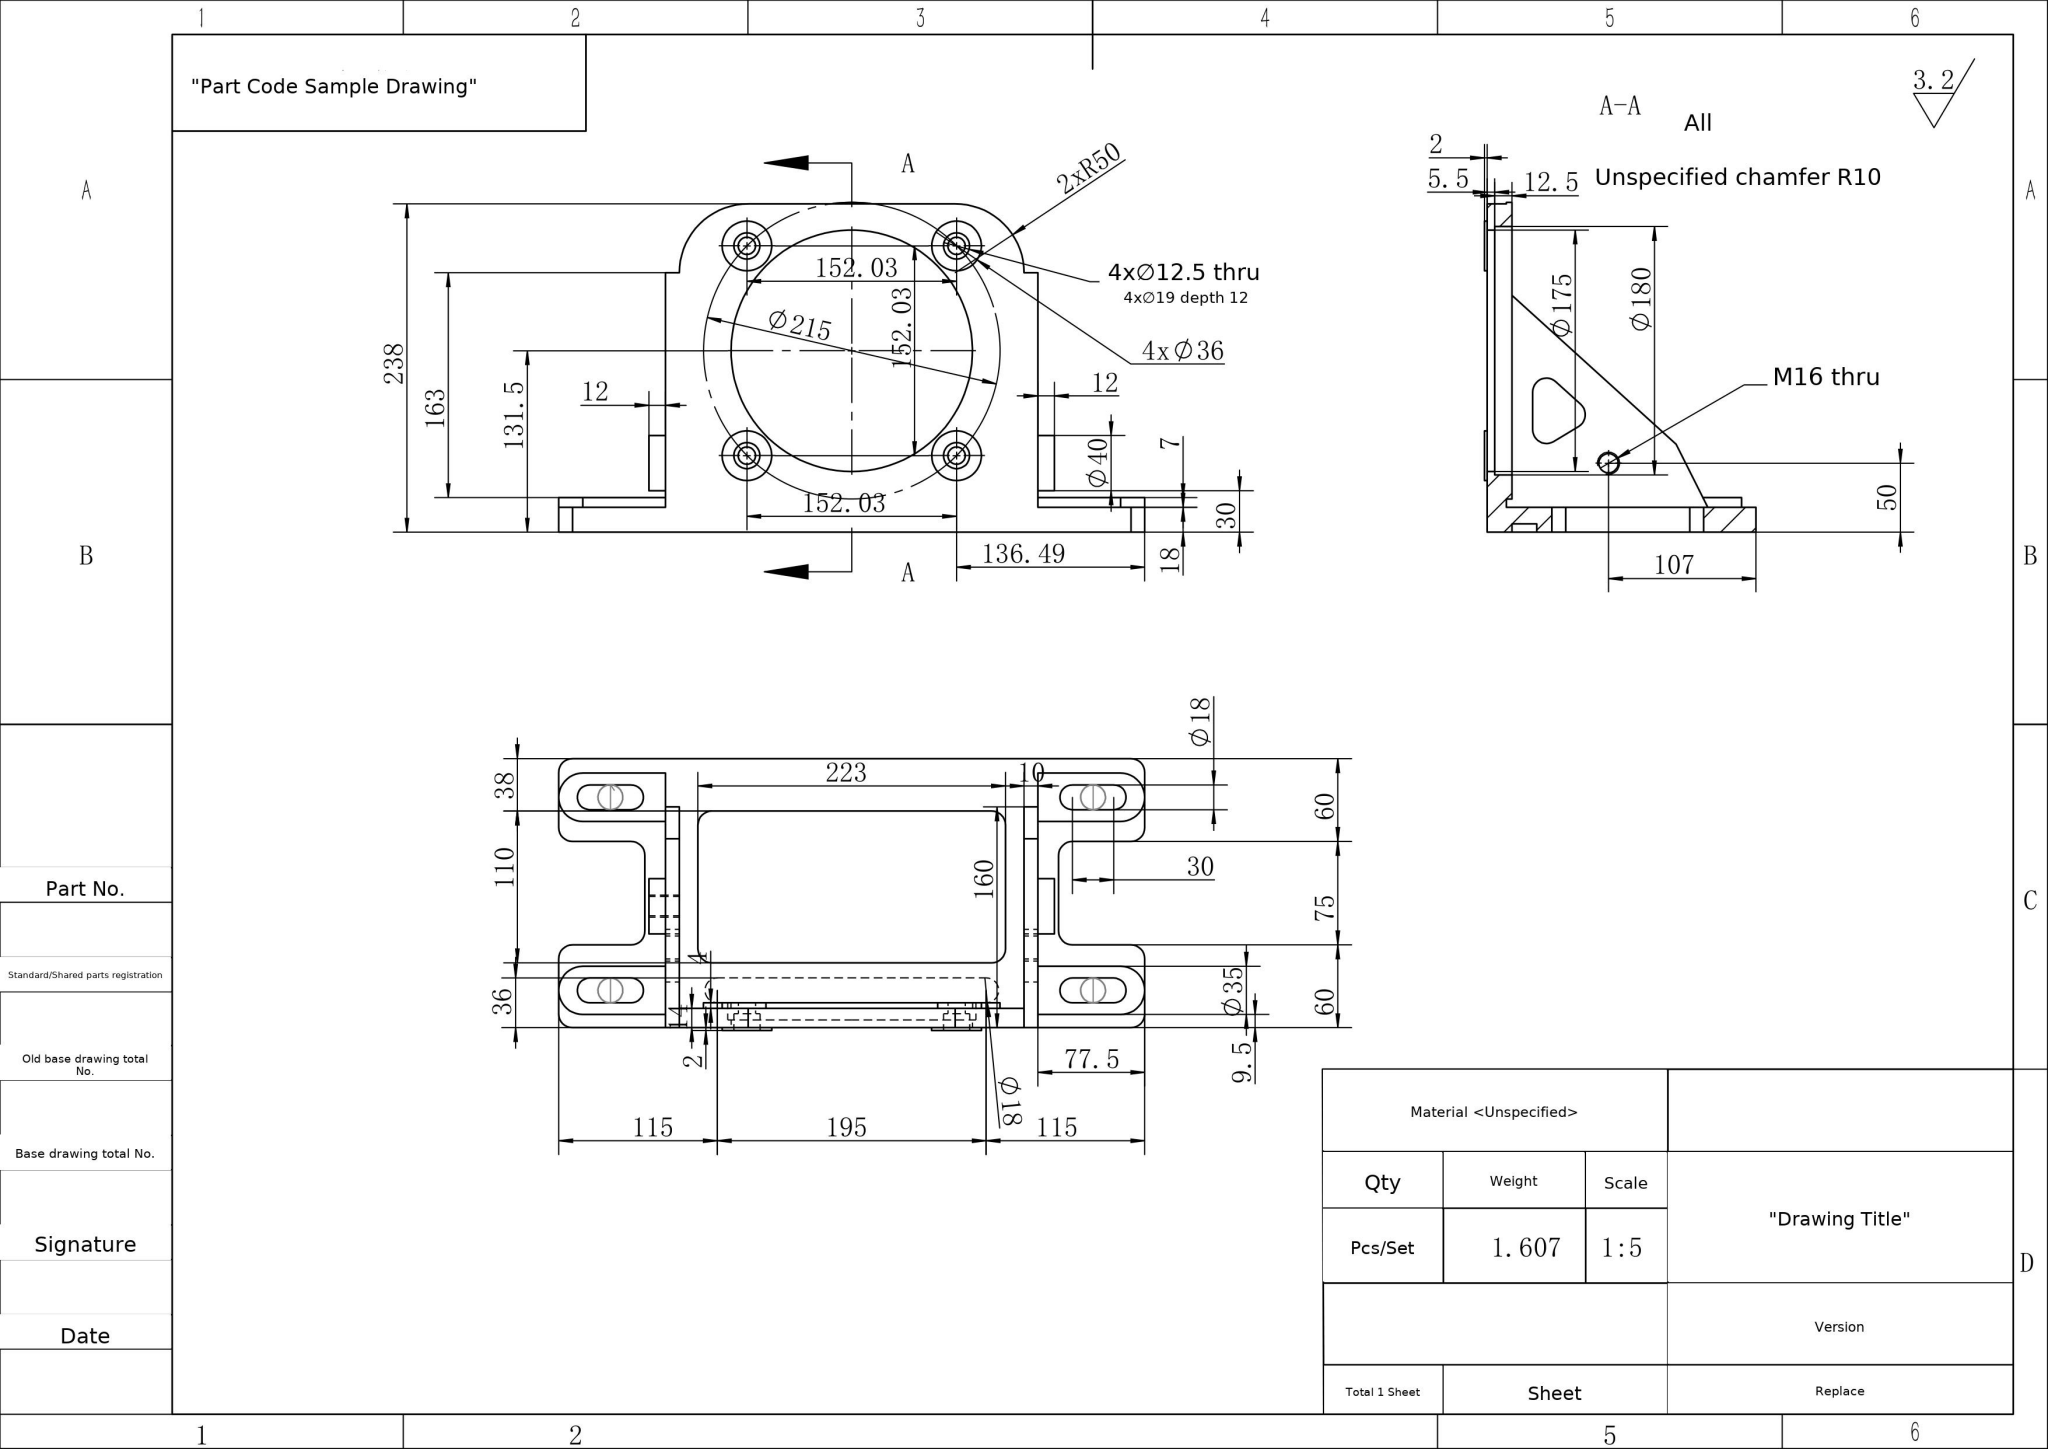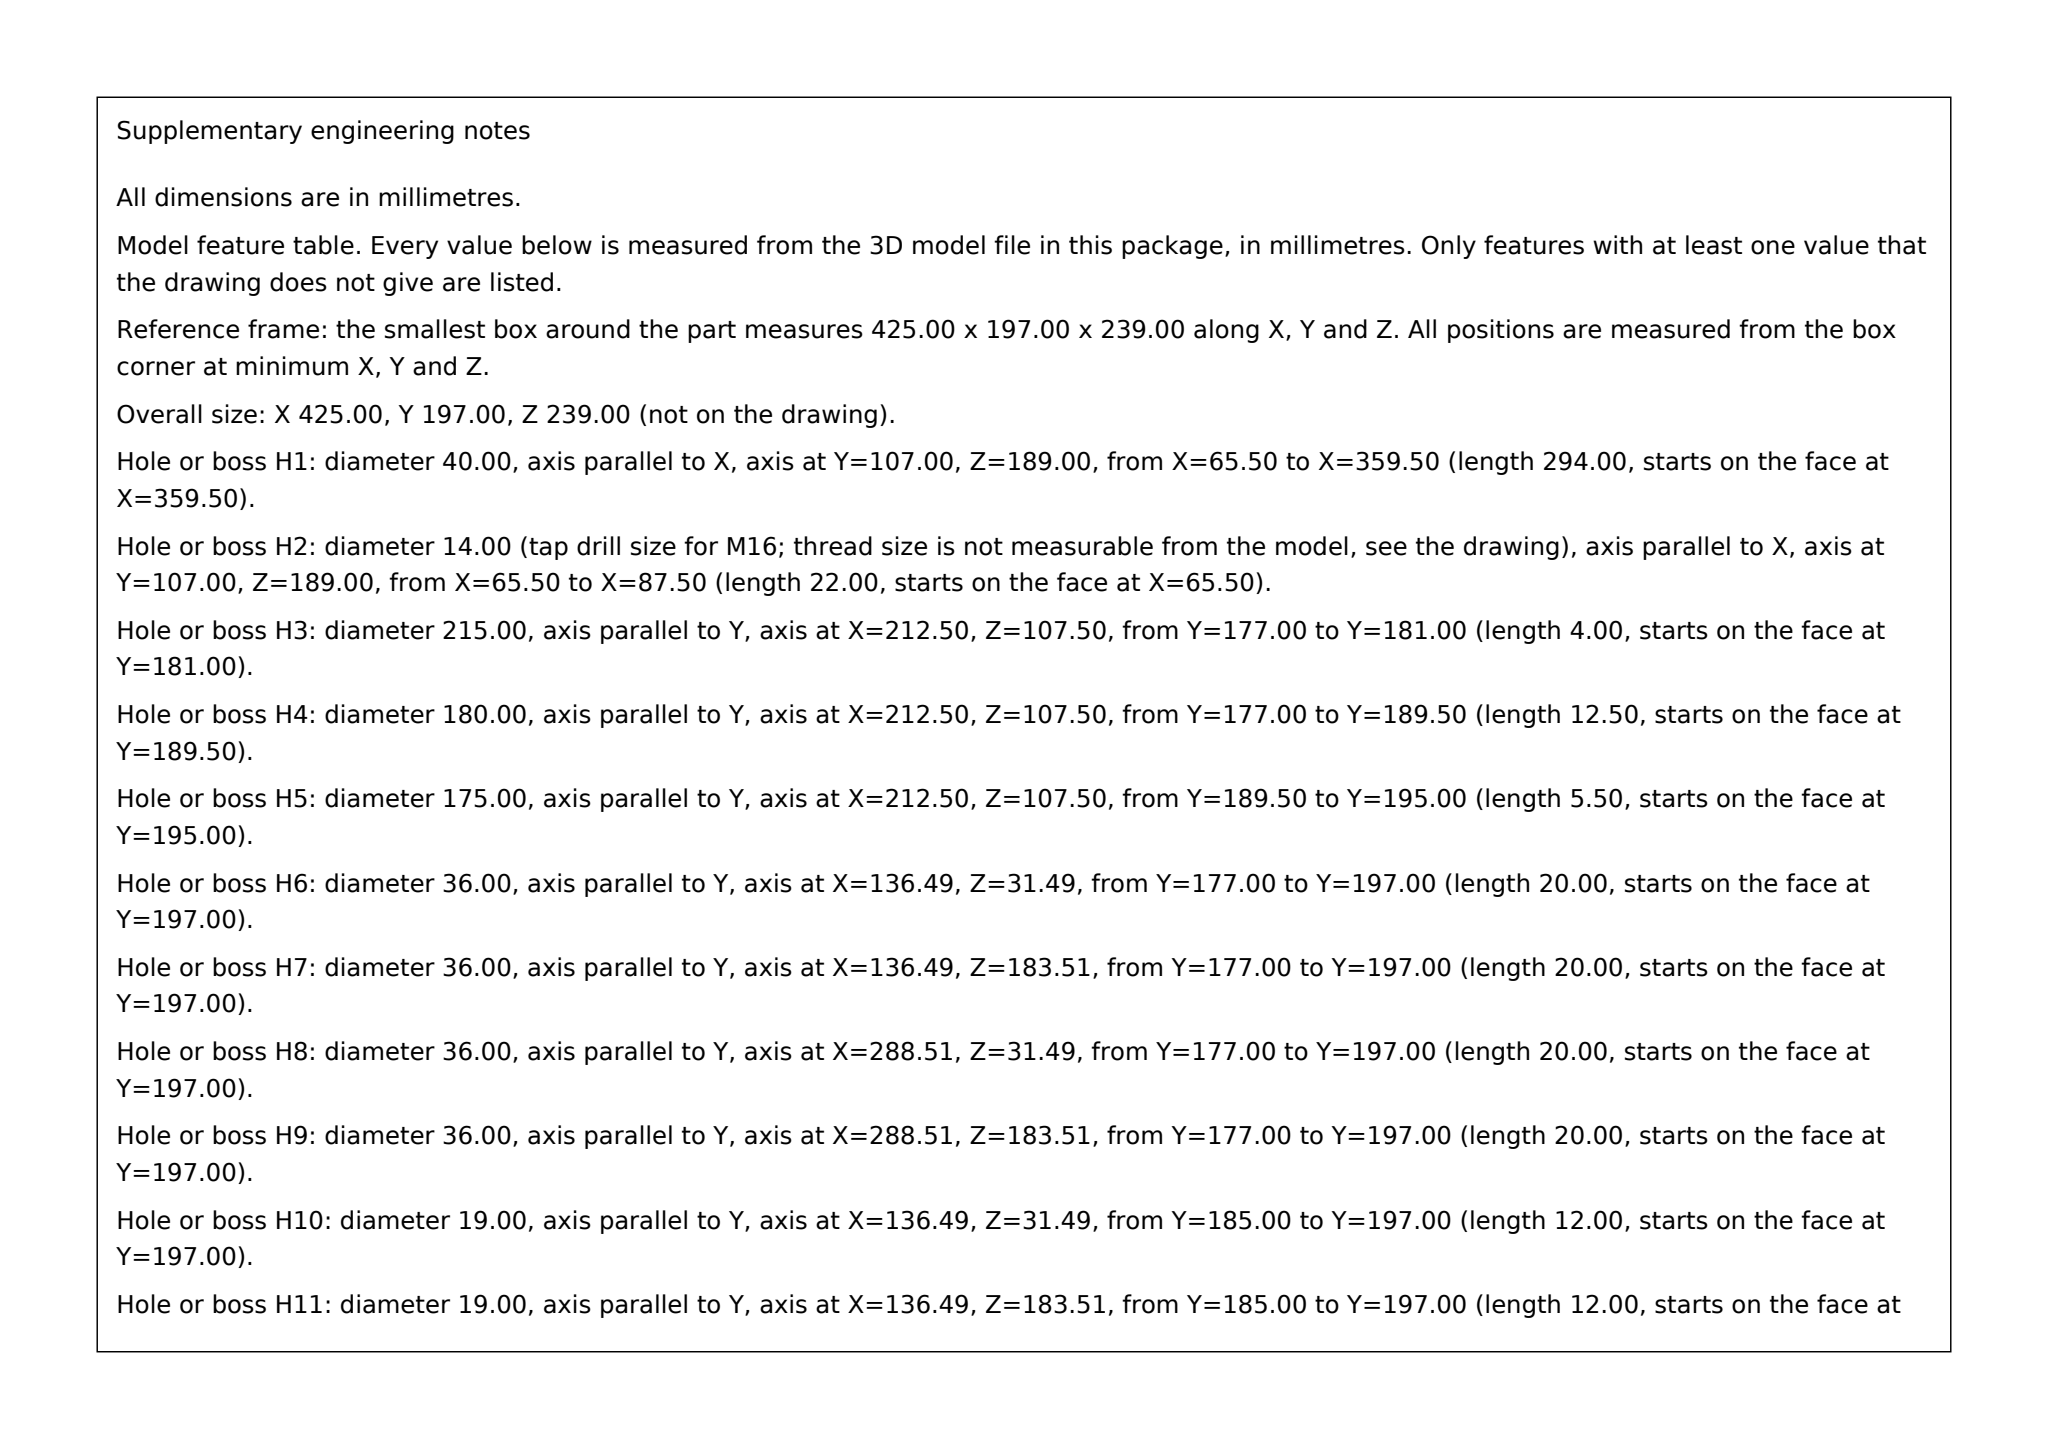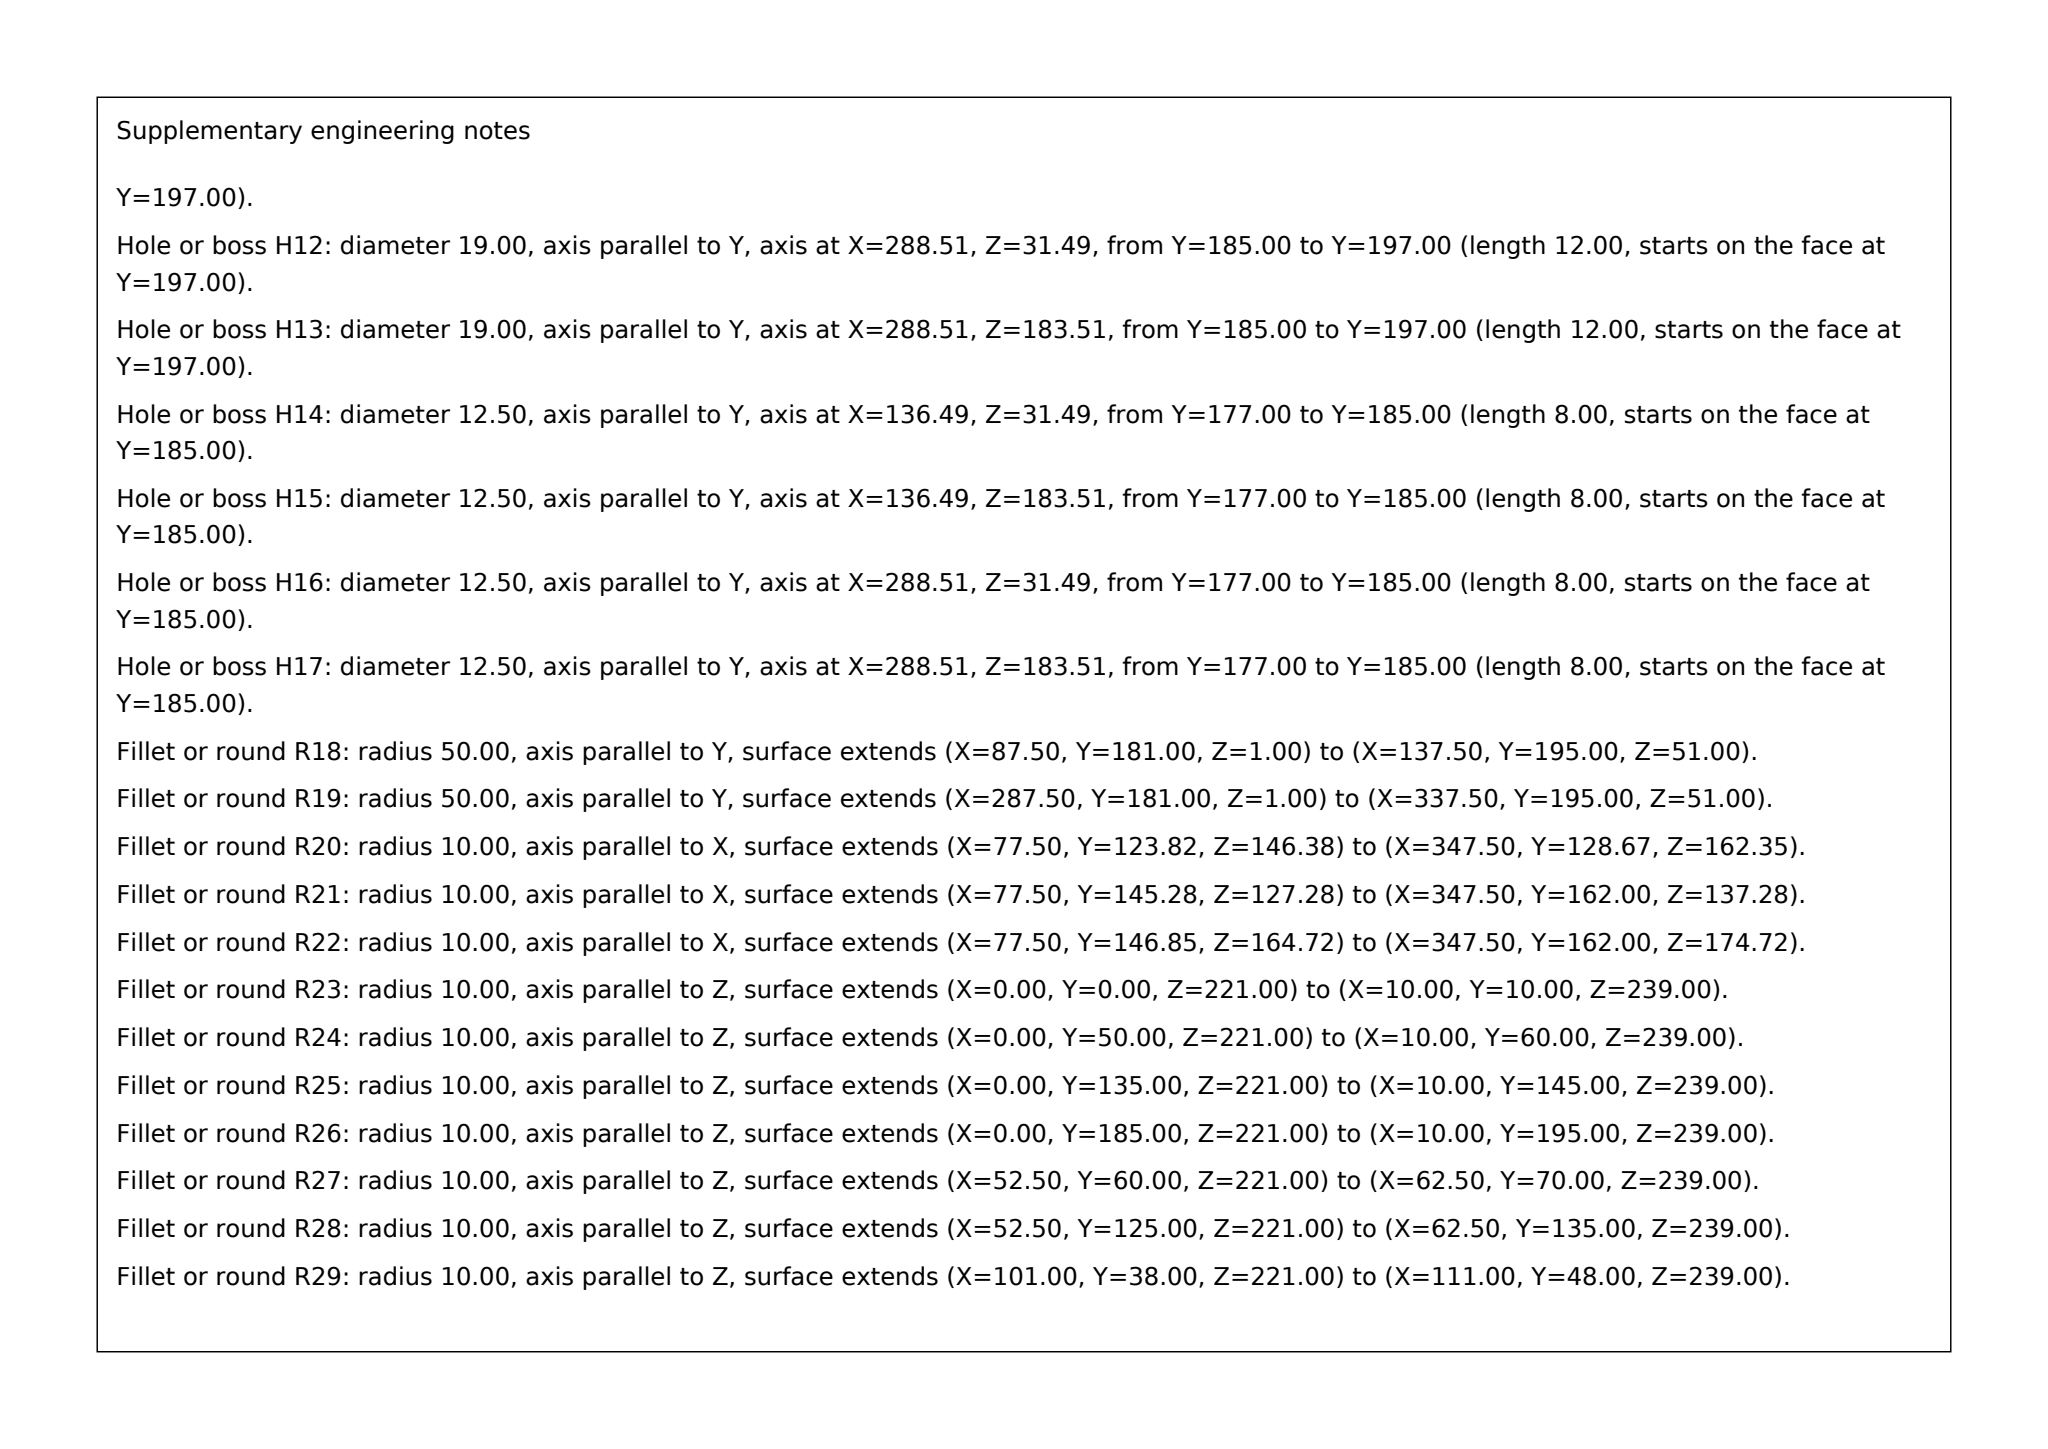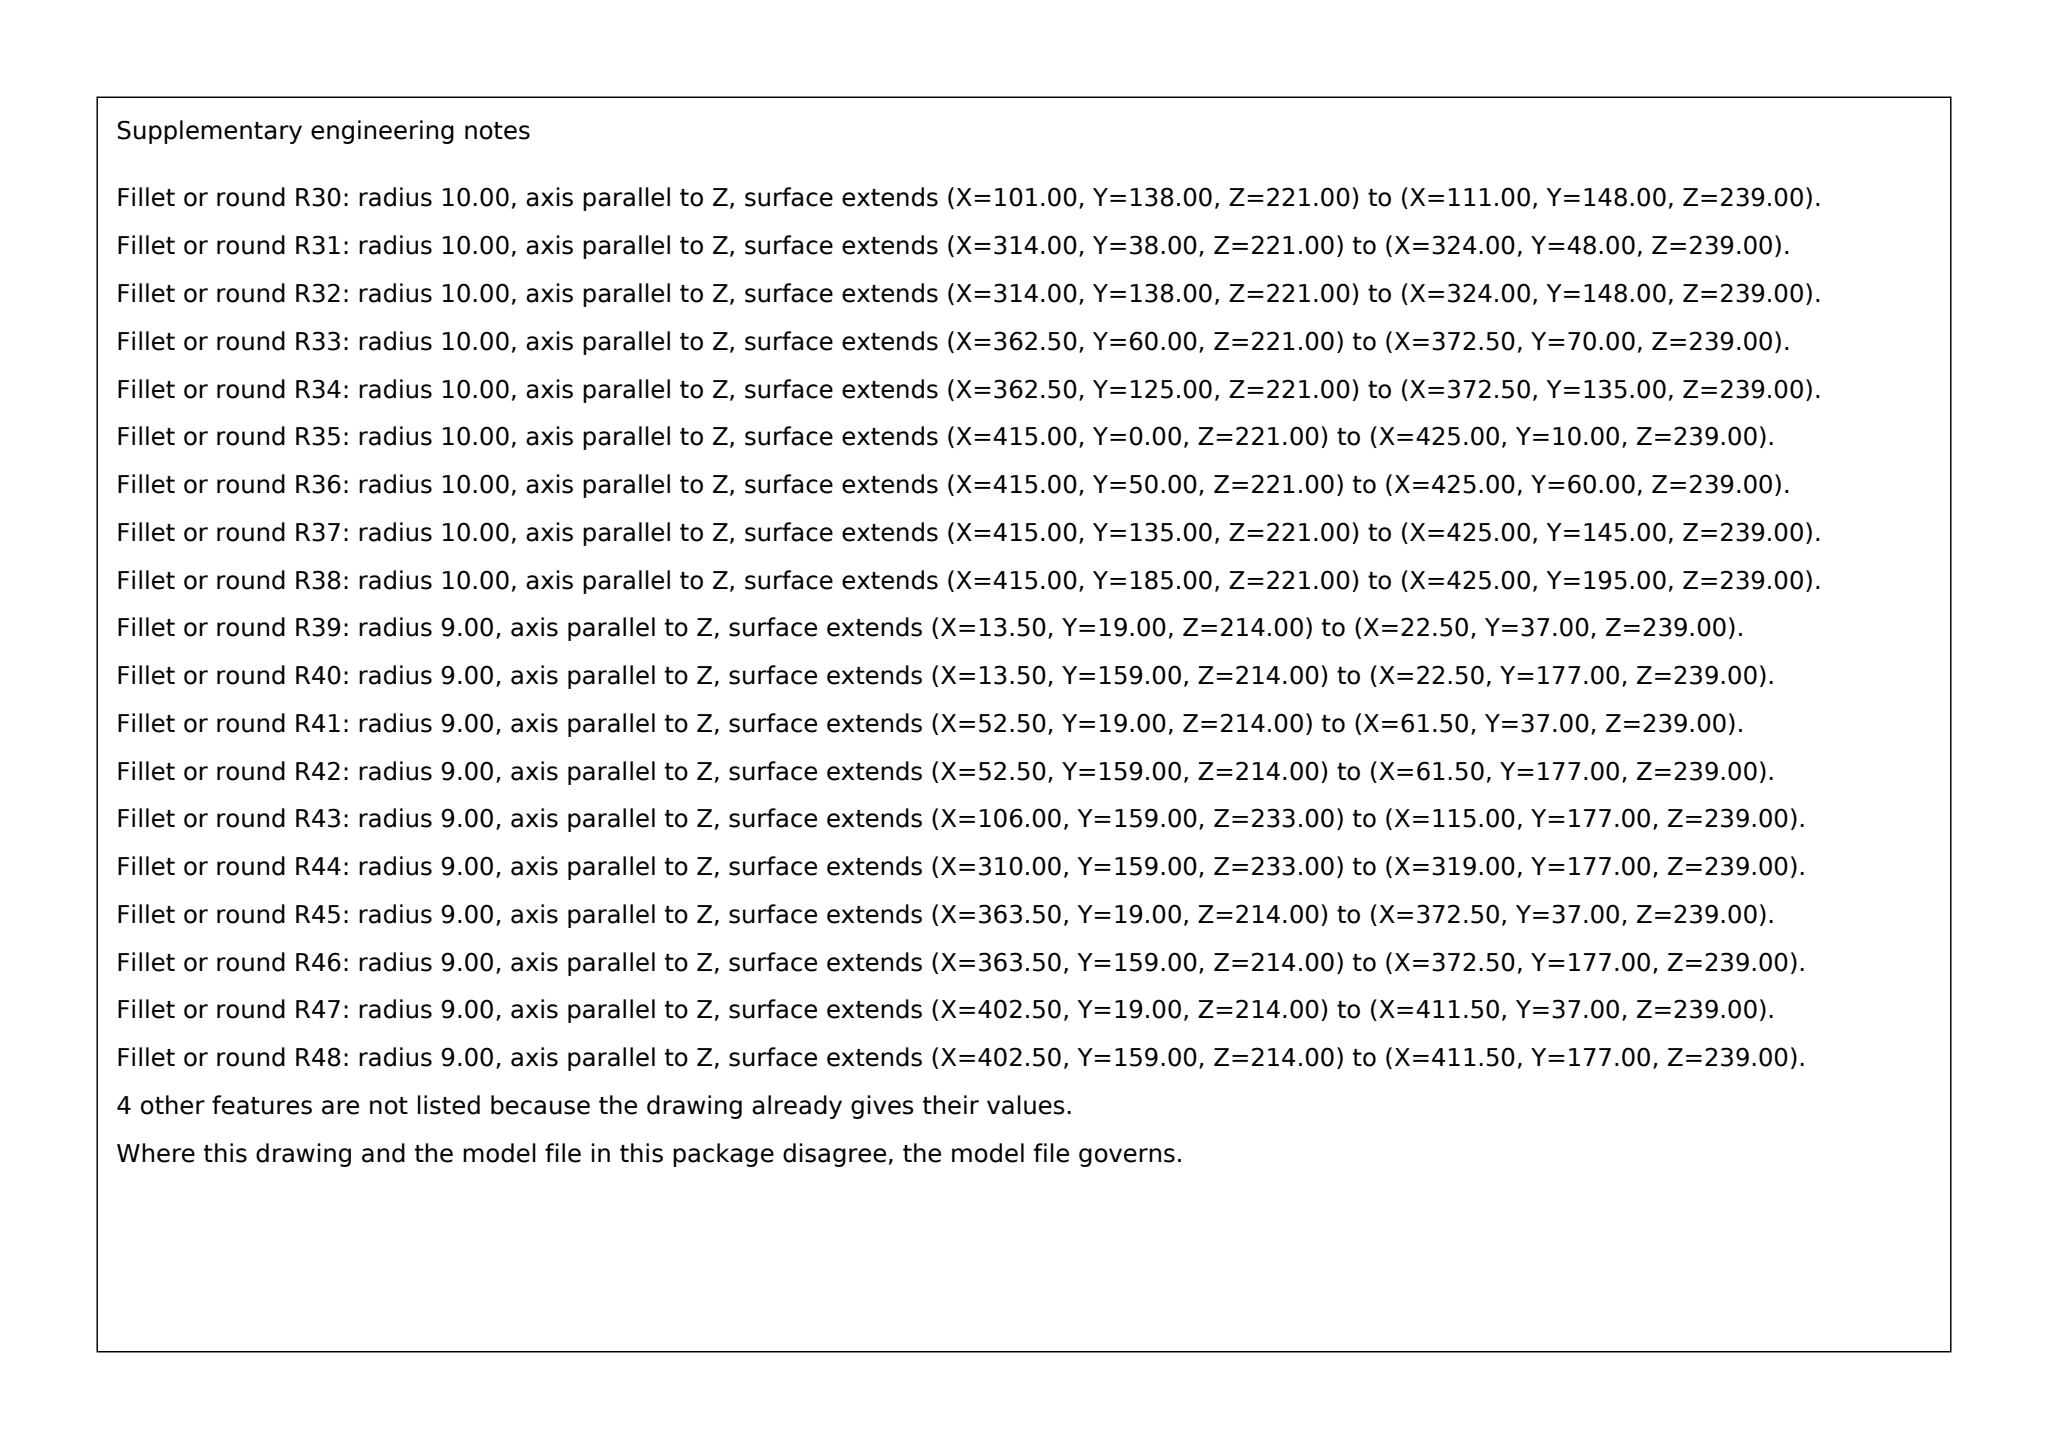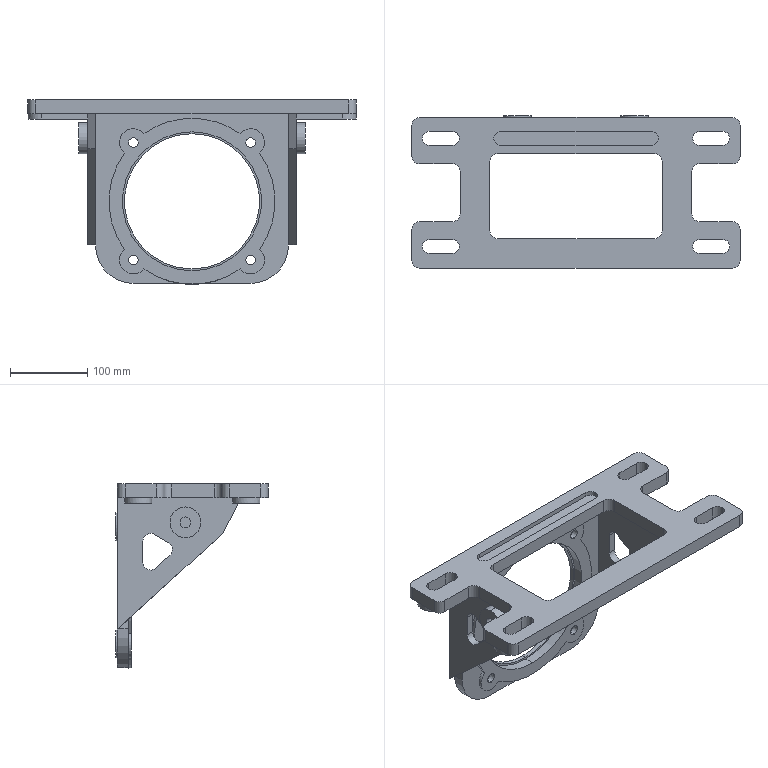Part | SolidWorks | mm | 1 solid | 170 faces | box 425 x 197 x 239 mm | volume 1607400 mm3 | cylinder 92 | plane 78 | commonest cylinder face diameters 20 x24 18 x15 36 x14 12.5 x8 19 x8 35 x6 215 x5 40 x4
build123d program:
from build123d import *

# Parameters (mm, degrees)
SKETCH1_W                    = 223
SKETCH1_H                    = 110
BOSS_EXTRUDE1_DEPTH          = 18
SKETCH2_W                    = 250
SKETCH2_H                    = 220
SKETCH2_R                    = 87.5
BOSS_EXTRUDE2_DEPTH          = 14
SKETCH3_R                    = 90
BOSS_EXTRUDE3_DEPTH          = 4
BOSS_EXTRUDE4_DEPTH          = 10
CUT_EXTRUDE1_START           = -8.5
SKETCH5_R                    = 90
CUT_EXTRUDE1_DEPTH           = 8.5
BOSS_EXTRUDE5_START          = 2
SKETCH6_R                    = 18
BOSS_EXTRUDE5_DEPTH          = 2
SKETCH7_R                    = 9.5
CUT_EXTRUDE2_DEPTH           = 12
F_12_5_12_5_DIAMETER_HOLE1_D = 12.5
BOSS_EXTRUDE6_DEPTH          = 7
FILLET1_R                    = 50
SKETCH11_R                   = 20
BOSS_EXTRUDE7_DEPTH          = 12
M16_TAPPED_HOLE1_D           = 14
M16_TAPPED_HOLE1_DEPTH       = 22
CUT_EXTRUDE4_DEPTH           = 424.671
FILLET2_R                    = 10
FILLET3_R                    = 10
CUT_EXTRUDE5_DEPTH           = 6
CUT_EXTRUDE6_DEPTH           = 335.929


with BuildPart() as part:
    # Sketch1 → Boss-Extrude1 (new body)
    with BuildSketch(Plane.XY):
        Polygon((-212.5, 97.5), (212.5, 97.5), (212.5, 37.5), (150, 37.5), (150, -37.5), (212.5, -37.5), (212.5, -97.5), (-212.5, -97.5), (-212.5, -37.5), (-150, -37.5), (-150, 37.5), (-212.5, 37.5), align=None)
        with Locations((0, -4.5)):
            Rectangle(SKETCH1_W, SKETCH1_H, mode=Mode.SUBTRACT)
    extrude(amount=BOSS_EXTRUDE1_DEPTH)

    # Sketch2 → Boss-Extrude2 (add)
    with BuildSketch(Plane(origin=(0, 97.5, 0), x_dir=(1, 0, 0), z_dir=(0, 1, 0))):
        with Locations((0, 110)):
            Rectangle(SKETCH2_W, SKETCH2_H)
        with Locations(Location((0, 113.5, 0), (0, 0, 270))):
            Circle(SKETCH2_R, mode=Mode.SUBTRACT)
    extrude(amount=-BOSS_EXTRUDE2_DEPTH)

    # Sketch3 → Boss-Extrude3 (add)
    with BuildSketch(Plane.XZ.offset(-83.5)):
        with BuildLine():
            ThreePointArc((87.632, -175.765), (107.5, -113.5), (87.632, -51.235))
            ThreePointArc((87.632, -51.235), (88.742, -24.758), (62.265, -25.868))
            ThreePointArc((62.265, -25.868), (0, -6), (-62.265, -25.868))
            ThreePointArc((-62.265, -25.868), (-88.742, -24.758), (-87.632, -51.235))
            ThreePointArc((-87.632, -51.235), (-107.5, -113.5), (-87.632, -175.765))
            ThreePointArc((-87.632, -175.765), (-88.742, -202.242), (-62.265, -201.132))
            ThreePointArc((-62.265, -201.132), (0, -221), (62.265, -201.132))
            ThreePointArc((62.265, -201.132), (88.742, -202.242), (87.632, -175.765))
        make_face()
        with Locations(Location((0, -113.5, 0), (0, 0, 270))):
            Circle(SKETCH3_R, mode=Mode.SUBTRACT)
    extrude(amount=BOSS_EXTRUDE3_DEPTH)

    # Sketch4 → Boss-Extrude4 (add)
    with BuildSketch(Plane.ZY.offset(125)):
        Polygon((0, 83.5), (0, -62.5), (-45.676, -39.5), (-170, 97.5), (0, 97.5), align=None)
    boss_extrude4 = extrude(amount=BOSS_EXTRUDE4_DEPTH)

    # Mirror1: Boss-Extrude4 across plane
    add(boss_extrude4.mirror(Plane.ZY))

    # Sketch5 → Cut-Extrude1 (cut)
    with BuildSketch(Plane.XZ.offset(-83.5).offset(CUT_EXTRUDE1_START)):
        with Locations(Location((0, -113.5, 0), (0, 0, 270))):
            Circle(SKETCH5_R)
    extrude(amount=CUT_EXTRUDE1_DEPTH, mode=Mode.SUBTRACT)

    # Sketch6 → Boss-Extrude5 (add)
    with BuildSketch(Plane(origin=(0, 97.5, 0), x_dir=(1, 0, 0), z_dir=(0, 1, 0)).offset(BOSS_EXTRUDE5_START)):
        with Locations(Location((-76.014, 189.514, 0), (0, 0, 90))):
            Circle(SKETCH6_R)
        with Locations(Location((76.014, 189.514, 0), (0, 0, 90))):
            Circle(SKETCH6_R)
        with Locations(Location((76.014, 37.486, 0), (0, 0, 90))):
            Circle(SKETCH6_R)
        with Locations(Location((-76.014, 37.486, 0), (0, 0, 90))):
            Circle(SKETCH6_R)
    extrude(amount=-BOSS_EXTRUDE5_DEPTH)

    # Sketch7 → Cut-Extrude2 (cut)
    with BuildSketch(Plane(origin=(0, 99.5, 0), x_dir=(1, 0, 0), z_dir=(0, 1, 0))):
        with Locations(Location((-76.014, 189.514, 0), (0, 0, 270))):
            Circle(SKETCH7_R)
        with Locations(Location((76.014, 189.514, 0), (0, 0, 270))):
            Circle(SKETCH7_R)
        with Locations(Location((-76.014, 37.486, 0), (0, 0, 270))):
            Circle(SKETCH7_R)
        with Locations(Location((76.014, 37.486, 0), (0, 0, 270))):
            Circle(SKETCH7_R)
    extrude(amount=-CUT_EXTRUDE2_DEPTH, mode=Mode.SUBTRACT)

    # 12.5 _12.5_ Diameter Hole1 (through all)
    with Locations(Plane(origin=(0, 87.5, 0), x_dir=(1, 0, 0), z_dir=(0, 1, 0))):
        with Locations((-76.014, 189.514), (76.014, 189.514), (-76.014, 37.486), (76.014, 37.486)):
            Hole(F_12_5_12_5_DIAMETER_HOLE1_D / 2)

    # Sketch10 → Boss-Extrude6 (add)
    with BuildSketch(Plane(origin=(0, 0, 0), x_dir=(-1, 0, 0), z_dir=(0, 0, -1))):
        with BuildLine():
            Line((135, 88), (195, 88))
            ThreePointArc((195, 88), (212.5, 70.5), (195, 53))
            Line((195, 53), (135, 53))
            Line((135, 53), (135, 88))
        make_face()
        with BuildLine():
            Line((135, -87), (195, -87))
            ThreePointArc((195, -87), (212.5, -69.5), (195, -52))
            Line((195, -52), (135, -52))
            Line((135, -52), (135, -87))
        make_face()
        with BuildLine():
            Line((-135, -52), (-135, -87))
            Line((-135, -87), (-195, -87))
            ThreePointArc((-195, -87), (-212.5, -69.5), (-195, -52))
            Line((-195, -52), (-135, -52))
        make_face()
        with BuildLine():
            Line((-135, 53), (-195, 53))
            ThreePointArc((-195, 53), (-212.5, 70.5), (-195, 88))
            Line((-195, 88), (-135, 88))
            Line((-135, 88), (-135, 53))
        make_face()
    extrude(amount=BOSS_EXTRUDE6_DEPTH)

    # Fillet1
    fillet1_edges = [part.edges().sort_by_distance(p)[0] for p in [
        (-125, 90.5, -220),
        (125, 90.5, -220),
    ]]
    fillet(fillet1_edges, radius=FILLET1_R)

    # Sketch11 → Boss-Extrude7 (add)
    with BuildSketch(Plane(origin=(135, 0, 0), x_dir=(0, 0, -1), z_dir=(1, 0, 0))):
        with Locations((32, 9.5)):
            Circle(SKETCH11_R)
    boss_extrude7 = extrude(amount=BOSS_EXTRUDE7_DEPTH)

    # Mirror2: Boss-Extrude7 across plane
    add(boss_extrude7.mirror(Plane.ZY))

    # M16 Tapped Hole1
    with Locations(Plane(origin=(-147, 0, 0), x_dir=(0, 0, -1), z_dir=(-1, 0, 0))):
        with Locations((32, -9.5)):
            Hole(M16_TAPPED_HOLE1_D / 2, depth=M16_TAPPED_HOLE1_DEPTH)

    # Sketch14 → Cut-Extrude4 (cut, through all)
    with BuildSketch(Plane.ZY.offset(135)):
        with BuildLine():
            Line((-91.121, 47.78), (-74.621, 29.598))
            ThreePointArc((-74.621, 29.598), (-66.24, 26.366), (-58.646, 31.165))
            Line((-58.646, 31.165), (-47.714, 49.347))
            ThreePointArc((-47.714, 49.347), (-47.58, 59.423), (-56.284, 64.5))
            Line((-56.284, 64.5), (-83.716, 64.5))
            ThreePointArc((-83.716, 64.5), (-92.859, 58.55), (-91.121, 47.78))
        make_face()
    extrude(amount=-CUT_EXTRUDE4_DEPTH, mode=Mode.SUBTRACT)

    # Fillet2
    fillet2_edges = [part.edges().sort_by_distance(p)[0] for p in [
        (212.5, -97.5, 9),
        (-212.5, -97.5, 9),
        (-212.5, -37.5, 9),
        (-150, -37.5, 9),
        (-150, 37.5, 9),
        (-212.5, 37.5, 9),
        (-212.5, 97.5, 9),
        (212.5, 97.5, 9),
        (212.5, 37.5, 9),
        (150, 37.5, 9),
        (150, -37.5, 9),
        (212.5, -37.5, 9),
    ]]
    fillet(fillet2_edges, radius=FILLET2_R)

    # Fillet3
    fillet3_edges = [part.edges().sort_by_distance(p)[0] for p in [
        (111.5, -59.5, 9),
        (111.5, 50.5, 9),
        (-111.5, 50.5, 9),
        (-111.5, -59.5, 9),
    ]]
    fillet(fillet3_edges, radius=FILLET3_R)

    # Sketch15 → Cut-Extrude5 (cut)
    with BuildSketch(Plane.XY.offset(18)):
        with BuildLine():
            Line((97.5, 61.5), (-97.5, 61.5))
            ThreePointArc((-97.5, 61.5), (-106.5, 70.5), (-97.5, 79.5))
            Line((-97.5, 79.5), (97.5, 79.5))
            ThreePointArc((97.5, 79.5), (106.5, 70.5), (97.5, 61.5))
        make_face()
    extrude(amount=-CUT_EXTRUDE5_DEPTH, mode=Mode.SUBTRACT)

    # Sketch16 → Cut-Extrude6 (cut, through all)
    with BuildSketch(Plane.XY.offset(18)):
        with BuildLine():
            Line((-190, 79.5), (-160, 79.5))
            ThreePointArc((-160, 79.5), (-151, 70.5), (-160, 61.5))
            Line((-160, 61.5), (-190, 61.5))
            ThreePointArc((-190, 61.5), (-199, 70.5), (-190, 79.5))
        make_face()
        with BuildLine():
            Line((160, 79.5), (190, 79.5))
            ThreePointArc((190, 79.5), (199, 70.5), (190, 61.5))
            Line((190, 61.5), (160, 61.5))
            ThreePointArc((160, 61.5), (151, 70.5), (160, 79.5))
        make_face()
        with BuildLine():
            Line((-190, -60.5), (-160, -60.5))
            ThreePointArc((-160, -60.5), (-151, -69.5), (-160, -78.5))
            Line((-160, -78.5), (-190, -78.5))
            ThreePointArc((-190, -78.5), (-199, -69.5), (-190, -60.5))
        make_face()
        with BuildLine():
            Line((160, -60.5), (190, -60.5))
            ThreePointArc((190, -60.5), (199, -69.5), (190, -78.5))
            Line((190, -78.5), (160, -78.5))
            ThreePointArc((160, -78.5), (151, -69.5), (160, -60.5))
        make_face()
    extrude(amount=-CUT_EXTRUDE6_DEPTH, mode=Mode.SUBTRACT)


solid = part.part